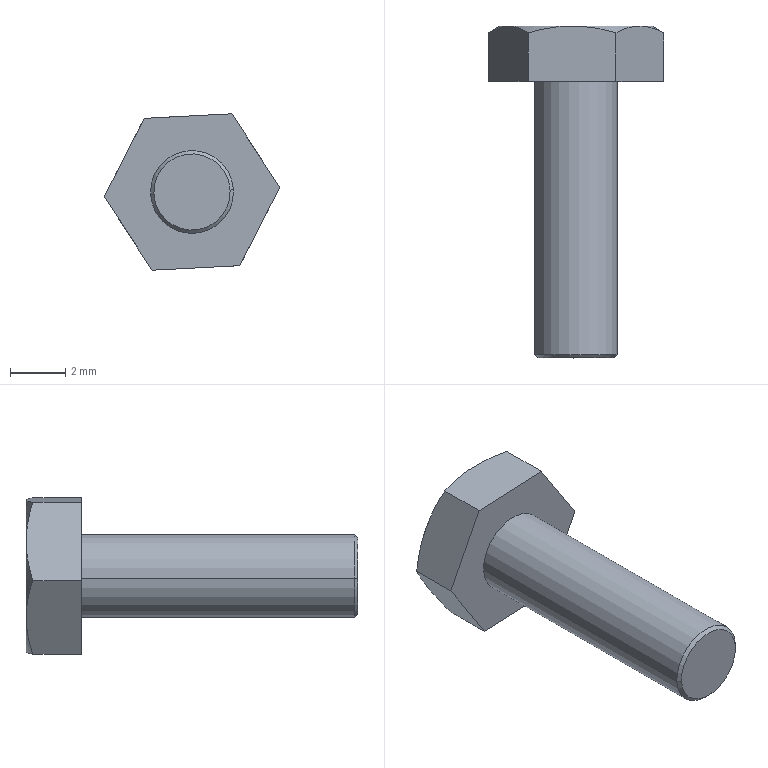Component | SolidWorks | TRCBASHexagonThroughHoleBolt[TRCBAS3-10]-1 | 1 solid | 20 faces | box 6.34 x 12 x 5.66 mm | volume 123 mm3 | cone 9 | plane 9 | cylinder 2 | commonest cylinder face diameters 3 x2
STEP:
#1=COLOUR_RGB('',0.7922,0.8196,0.9333);
#2=FILL_AREA_STYLE_COLOUR('',#1);
#3=FILL_AREA_STYLE('',(#2));
#4=SURFACE_STYLE_FILL_AREA(#3);
#5=SURFACE_SIDE_STYLE('',(#4));
#6=SURFACE_STYLE_USAGE(.BOTH.,#5);
#7=PRESENTATION_STYLE_ASSIGNMENT((#6));
#8=CARTESIAN_POINT('',(2.505,-3.607,-10.617));
#9=VERTEX_POINT('',#8);
#10=CARTESIAN_POINT('',(2.397,-3.607,-10.623));
#11=VERTEX_POINT('',#10);
#12=CARTESIAN_POINT('',(2.451,-3.607,-10.62));
#13=DIRECTION('',(0.,-1.,-0.));
#14=DIRECTION('',(0.9987,0.,0.05162));
#15=AXIS2_PLACEMENT_3D('',#12,#13,#14);
#16=CIRCLE('',#15,0.05433);
#17=EDGE_CURVE('',#9,#11,#16,.T.);
#18=ORIENTED_EDGE('',*,*,#17,.F.);
#19=CARTESIAN_POINT('',(2.51,-3.602,-10.617));
#20=VERTEX_POINT('',#19);
#21=CARTESIAN_POINT('',(2.51,-3.602,-10.617));
#22=DIRECTION('',(0.7062,0.7071,0.0365));
#23=VECTOR('',#22,39.37);
#24=LINE('',#21,#23);
#25=EDGE_CURVE('',#9,#20,#24,.T.);
#26=ORIENTED_EDGE('',*,*,#25,.T.);
#27=CARTESIAN_POINT('',(2.392,-3.602,-10.623));
#28=VERTEX_POINT('',#27);
#29=CARTESIAN_POINT('',(2.451,-3.602,-10.62));
#30=DIRECTION('',(-0.,1.,-0.));
#31=DIRECTION('',(0.9987,0.,0.05162));
#32=AXIS2_PLACEMENT_3D('',#29,#30,#31);
#33=CIRCLE('',#32,0.05906);
#34=EDGE_CURVE('',#28,#20,#33,.T.);
#35=ORIENTED_EDGE('',*,*,#34,.F.);
#36=CARTESIAN_POINT('',(2.392,-3.602,-10.623));
#37=DIRECTION('',(-0.7062,0.7071,-0.0365));
#38=VECTOR('',#37,39.37);
#39=LINE('',#36,#38);
#40=EDGE_CURVE('',#11,#28,#39,.T.);
#41=ORIENTED_EDGE('',*,*,#40,.F.);
#42=EDGE_LOOP('',(#18,#26,#35,#41));
#43=FACE_OUTER_BOUND('',#42,.T.);
#44=CARTESIAN_POINT('',(2.451,-3.602,-10.62));
#45=DIRECTION('',(-0.,1.,-0.));
#46=DIRECTION('',(-0.9987,0.,-0.05162));
#47=AXIS2_PLACEMENT_3D('',#44,#45,#46);
#48=CONICAL_SURFACE('',#47,0.05906,0.7854);
#49=ADVANCED_FACE('',(#43),#48,.T.);
#50=CARTESIAN_POINT('',(2.559,-3.134,-10.614));
#51=VERTEX_POINT('',#50);
#52=CARTESIAN_POINT('',(2.547,-3.134,-10.669));
#53=VERTEX_POINT('',#52);
#54=CARTESIAN_POINT('',(2.451,-3.134,-10.62));
#55=DIRECTION('',(-0.,1.,0.));
#56=DIRECTION('',(-0.9987,0.,-0.05162));
#57=AXIS2_PLACEMENT_3D('',#54,#55,#56);
#58=CIRCLE('',#57,0.1083);
#59=EDGE_CURVE('',#51,#53,#58,.T.);
#60=ORIENTED_EDGE('',*,*,#59,.F.);
#61=CARTESIAN_POINT('',(2.576,-3.144,-10.614));
#62=VERTEX_POINT('',#61);
#63=CARTESIAN_POINT('',(2.559,-3.134,-10.614));
#64=DIRECTION('',(0.8649,-0.5,0.0447));
#65=VECTOR('',#64,39.37);
#66=LINE('',#63,#65);
#67=EDGE_CURVE('',#51,#62,#66,.T.);
#68=ORIENTED_EDGE('',*,*,#67,.T.);
#69=CARTESIAN_POINT('',(2.547,-3.134,-10.669));
#70=CARTESIAN_POINT('',(2.552,-3.134,-10.66));
#71=CARTESIAN_POINT('',(2.557,-3.135,-10.65));
#72=CARTESIAN_POINT('',(2.567,-3.138,-10.632));
#73=CARTESIAN_POINT('',(2.571,-3.141,-10.623));
#74=CARTESIAN_POINT('',(2.576,-3.144,-10.614));
#75=B_SPLINE_CURVE_WITH_KNOTS('',3,(#69,#70,#71,#72,#73,#74),.UNSPECIFIED.,.F.,.F.,(4,2,4),(0.001607,0.002407,0.003207),.UNSPECIFIED.);
#76=EDGE_CURVE('',#53,#62,#75,.T.);
#77=ORIENTED_EDGE('',*,*,#76,.F.);
#78=EDGE_LOOP('',(#60,#68,#77));
#79=FACE_OUTER_BOUND('',#78,.T.);
#80=CARTESIAN_POINT('',(2.451,-3.134,-10.62));
#81=DIRECTION('',(0.,-1.,-0.));
#82=DIRECTION('',(0.9987,0.,0.05162));
#83=AXIS2_PLACEMENT_3D('',#80,#81,#82);
#84=CONICAL_SURFACE('',#83,0.1083,1.047);
#85=ADVANCED_FACE('',(#79),#84,.T.);
#86=ORIENTED_EDGE('',*,*,#34,.T.);
#87=CARTESIAN_POINT('',(2.51,-3.213,-10.617));
#88=VERTEX_POINT('',#87);
#89=CARTESIAN_POINT('',(2.51,-3.134,-10.617));
#90=DIRECTION('',(-0.,1.,0.));
#91=VECTOR('',#90,39.37);
#92=LINE('',#89,#91);
#93=EDGE_CURVE('',#20,#88,#92,.T.);
#94=ORIENTED_EDGE('',*,*,#93,.T.);
#95=CARTESIAN_POINT('',(2.392,-3.213,-10.623));
#96=VERTEX_POINT('',#95);
#97=CARTESIAN_POINT('',(2.451,-3.213,-10.62));
#98=DIRECTION('',(-0.,1.,0.));
#99=DIRECTION('',(-0.9987,0.,-0.05162));
#100=AXIS2_PLACEMENT_3D('',#97,#98,#99);
#101=CIRCLE('',#100,0.05906);
#102=EDGE_CURVE('',#96,#88,#101,.T.);
#103=ORIENTED_EDGE('',*,*,#102,.F.);
#104=CARTESIAN_POINT('',(2.392,-3.134,-10.623));
#105=DIRECTION('',(-0.,1.,0.));
#106=VECTOR('',#105,39.37);
#107=LINE('',#104,#106);
#108=EDGE_CURVE('',#28,#96,#107,.T.);
#109=ORIENTED_EDGE('',*,*,#108,.F.);
#110=EDGE_LOOP('',(#86,#94,#103,#109));
#111=FACE_OUTER_BOUND('',#110,.T.);
#112=CARTESIAN_POINT('',(2.451,-3.134,-10.62));
#113=DIRECTION('',(-0.,1.,0.));
#114=DIRECTION('',(-0.9987,0.,-0.05162));
#115=AXIS2_PLACEMENT_3D('',#112,#113,#114);
#116=CYLINDRICAL_SURFACE('',#115,0.05906);
#117=ADVANCED_FACE('',(#111),#116,.T.);
#118=CARTESIAN_POINT('',(2.576,-3.213,-10.614));
#119=VERTEX_POINT('',#118);
#120=CARTESIAN_POINT('',(2.576,-3.213,-10.614));
#121=DIRECTION('',(-0.,1.,0.));
#122=VECTOR('',#121,39.37);
#123=LINE('',#120,#122);
#124=EDGE_CURVE('',#119,#62,#123,.T.);
#125=ORIENTED_EDGE('',*,*,#124,.T.);
#126=CARTESIAN_POINT('',(2.542,-3.134,-10.561));
#127=VERTEX_POINT('',#126);
#128=CARTESIAN_POINT('',(2.576,-3.144,-10.614));
#129=CARTESIAN_POINT('',(2.565,-3.138,-10.596));
#130=CARTESIAN_POINT('',(2.553,-3.134,-10.579));
#131=CARTESIAN_POINT('',(2.542,-3.134,-10.561));
#132=B_SPLINE_CURVE_WITH_KNOTS('',3,(#128,#129,#130,#131),.UNSPECIFIED.,.F.,.F.,(4,4),(0.00000024,0.001607),.UNSPECIFIED.);
#133=EDGE_CURVE('',#62,#127,#132,.T.);
#134=ORIENTED_EDGE('',*,*,#133,.T.);
#135=CARTESIAN_POINT('',(2.508,-3.144,-10.509));
#136=VERTEX_POINT('',#135);
#137=CARTESIAN_POINT('',(2.542,-3.134,-10.561));
#138=CARTESIAN_POINT('',(2.536,-3.134,-10.552));
#139=CARTESIAN_POINT('',(2.53,-3.135,-10.543));
#140=CARTESIAN_POINT('',(2.519,-3.138,-10.526));
#141=CARTESIAN_POINT('',(2.513,-3.141,-10.517));
#142=CARTESIAN_POINT('',(2.508,-3.144,-10.509));
#143=B_SPLINE_CURVE_WITH_KNOTS('',3,(#137,#138,#139,#140,#141,#142),.UNSPECIFIED.,.F.,.F.,(4,2,4),(0.001607,0.002407,0.003207),.UNSPECIFIED.);
#144=EDGE_CURVE('',#127,#136,#143,.T.);
#145=ORIENTED_EDGE('',*,*,#144,.T.);
#146=CARTESIAN_POINT('',(2.508,-3.213,-10.509));
#147=VERTEX_POINT('',#146);
#148=CARTESIAN_POINT('',(2.508,-3.213,-10.509));
#149=DIRECTION('',(-0.,1.,0.));
#150=VECTOR('',#149,39.37);
#151=LINE('',#148,#150);
#152=EDGE_CURVE('',#147,#136,#151,.T.);
#153=ORIENTED_EDGE('',*,*,#152,.F.);
#154=CARTESIAN_POINT('',(2.508,-3.213,-10.509));
#155=DIRECTION('',(0.544,0.,-0.8391));
#156=VECTOR('',#155,39.37);
#157=LINE('',#154,#156);
#158=EDGE_CURVE('',#147,#119,#157,.T.);
#159=ORIENTED_EDGE('',*,*,#158,.T.);
#160=EDGE_LOOP('',(#125,#134,#145,#153,#159));
#161=FACE_OUTER_BOUND('',#160,.T.);
#162=CARTESIAN_POINT('',(2.508,-3.213,-10.509));
#163=DIRECTION('',(0.8391,0.,0.544));
#164=DIRECTION('',(0.544,0.,-0.8391));
#165=AXIS2_PLACEMENT_3D('',#162,#163,#164);
#166=PLANE('',#165);
#167=ADVANCED_FACE('',(#161),#166,.T.);
#168=ORIENTED_EDGE('',*,*,#152,.T.);
#169=CARTESIAN_POINT('',(2.445,-3.134,-10.512));
#170=VERTEX_POINT('',#169);
#171=CARTESIAN_POINT('',(2.508,-3.144,-10.509));
#172=CARTESIAN_POINT('',(2.498,-3.141,-10.509));
#173=CARTESIAN_POINT('',(2.488,-3.139,-10.51));
#174=CARTESIAN_POINT('',(2.467,-3.135,-10.511));
#175=CARTESIAN_POINT('',(2.456,-3.134,-10.511));
#176=CARTESIAN_POINT('',(2.445,-3.134,-10.512));
#177=B_SPLINE_CURVE_WITH_KNOTS('',3,(#171,#172,#173,#174,#175,#176),.UNSPECIFIED.,.F.,.F.,(4,2,4),(0.008159,0.008963,0.009767),.UNSPECIFIED.);
#178=EDGE_CURVE('',#136,#170,#177,.T.);
#179=ORIENTED_EDGE('',*,*,#178,.T.);
#180=CARTESIAN_POINT('',(2.383,-3.144,-10.515));
#181=VERTEX_POINT('',#180);
#182=CARTESIAN_POINT('',(2.445,-3.134,-10.512));
#183=CARTESIAN_POINT('',(2.435,-3.134,-10.513));
#184=CARTESIAN_POINT('',(2.424,-3.135,-10.513));
#185=CARTESIAN_POINT('',(2.404,-3.138,-10.514));
#186=CARTESIAN_POINT('',(2.393,-3.141,-10.515));
#187=CARTESIAN_POINT('',(2.383,-3.144,-10.515));
#188=B_SPLINE_CURVE_WITH_KNOTS('',3,(#182,#183,#184,#185,#186,#187),.UNSPECIFIED.,.F.,.F.,(4,2,4),(0.009767,0.01057,0.01137),.UNSPECIFIED.);
#189=EDGE_CURVE('',#170,#181,#188,.T.);
#190=ORIENTED_EDGE('',*,*,#189,.T.);
#191=CARTESIAN_POINT('',(2.383,-3.213,-10.515));
#192=VERTEX_POINT('',#191);
#193=CARTESIAN_POINT('',(2.383,-3.213,-10.515));
#194=DIRECTION('',(-0.,1.,0.));
#195=VECTOR('',#194,39.37);
#196=LINE('',#193,#195);
#197=EDGE_CURVE('',#192,#181,#196,.T.);
#198=ORIENTED_EDGE('',*,*,#197,.F.);
#199=CARTESIAN_POINT('',(2.383,-3.213,-10.515));
#200=DIRECTION('',(0.9987,0.,0.05162));
#201=VECTOR('',#200,39.37);
#202=LINE('',#199,#201);
#203=EDGE_CURVE('',#192,#147,#202,.T.);
#204=ORIENTED_EDGE('',*,*,#203,.T.);
#205=EDGE_LOOP('',(#168,#179,#190,#198,#204));
#206=FACE_OUTER_BOUND('',#205,.T.);
#207=CARTESIAN_POINT('',(2.383,-3.213,-10.515));
#208=DIRECTION('',(-0.05162,-0.,0.9987));
#209=DIRECTION('',(0.9987,-0.,0.05162));
#210=AXIS2_PLACEMENT_3D('',#207,#208,#209);
#211=PLANE('',#210);
#212=ADVANCED_FACE('',(#206),#211,.T.);
#213=ORIENTED_EDGE('',*,*,#197,.T.);
#214=CARTESIAN_POINT('',(2.355,-3.134,-10.571));
#215=VERTEX_POINT('',#214);
#216=CARTESIAN_POINT('',(2.383,-3.144,-10.515));
#217=CARTESIAN_POINT('',(2.374,-3.138,-10.533));
#218=CARTESIAN_POINT('',(2.364,-3.134,-10.552));
#219=CARTESIAN_POINT('',(2.355,-3.134,-10.571));
#220=B_SPLINE_CURVE_WITH_KNOTS('',3,(#216,#217,#218,#219),.UNSPECIFIED.,.F.,.F.,(4,4),(0.00000024,0.001607),.UNSPECIFIED.);
#221=EDGE_CURVE('',#181,#215,#220,.T.);
#222=ORIENTED_EDGE('',*,*,#221,.T.);
#223=CARTESIAN_POINT('',(2.326,-3.144,-10.627));
#224=VERTEX_POINT('',#223);
#225=CARTESIAN_POINT('',(2.355,-3.134,-10.571));
#226=CARTESIAN_POINT('',(2.35,-3.134,-10.58));
#227=CARTESIAN_POINT('',(2.345,-3.135,-10.59));
#228=CARTESIAN_POINT('',(2.336,-3.138,-10.608));
#229=CARTESIAN_POINT('',(2.331,-3.141,-10.617));
#230=CARTESIAN_POINT('',(2.326,-3.144,-10.627));
#231=B_SPLINE_CURVE_WITH_KNOTS('',3,(#225,#226,#227,#228,#229,#230),.UNSPECIFIED.,.F.,.F.,(4,2,4),(0.001607,0.002407,0.003207),.UNSPECIFIED.);
#232=EDGE_CURVE('',#215,#224,#231,.T.);
#233=ORIENTED_EDGE('',*,*,#232,.T.);
#234=CARTESIAN_POINT('',(2.326,-3.213,-10.627));
#235=VERTEX_POINT('',#234);
#236=CARTESIAN_POINT('',(2.326,-3.213,-10.627));
#237=DIRECTION('',(-0.,1.,0.));
#238=VECTOR('',#237,39.37);
#239=LINE('',#236,#238);
#240=EDGE_CURVE('',#235,#224,#239,.T.);
#241=ORIENTED_EDGE('',*,*,#240,.F.);
#242=CARTESIAN_POINT('',(2.326,-3.213,-10.627));
#243=DIRECTION('',(0.4546,0.,0.8907));
#244=VECTOR('',#243,39.37);
#245=LINE('',#242,#244);
#246=EDGE_CURVE('',#235,#192,#245,.T.);
#247=ORIENTED_EDGE('',*,*,#246,.T.);
#248=EDGE_LOOP('',(#213,#222,#233,#241,#247));
#249=FACE_OUTER_BOUND('',#248,.T.);
#250=CARTESIAN_POINT('',(2.326,-3.213,-10.627));
#251=DIRECTION('',(-0.8907,-0.,0.4546));
#252=DIRECTION('',(0.4546,-0.,0.8907));
#253=AXIS2_PLACEMENT_3D('',#250,#251,#252);
#254=PLANE('',#253);
#255=ADVANCED_FACE('',(#249),#254,.T.);
#256=ORIENTED_EDGE('',*,*,#240,.T.);
#257=CARTESIAN_POINT('',(2.36,-3.134,-10.679));
#258=VERTEX_POINT('',#257);
#259=CARTESIAN_POINT('',(2.326,-3.144,-10.627));
#260=CARTESIAN_POINT('',(2.337,-3.138,-10.644));
#261=CARTESIAN_POINT('',(2.349,-3.134,-10.661));
#262=CARTESIAN_POINT('',(2.36,-3.134,-10.679));
#263=B_SPLINE_CURVE_WITH_KNOTS('',3,(#259,#260,#261,#262),.UNSPECIFIED.,.F.,.F.,(4,4),(0.00000024,0.001607),.UNSPECIFIED.);
#264=EDGE_CURVE('',#224,#258,#263,.T.);
#265=ORIENTED_EDGE('',*,*,#264,.T.);
#266=CARTESIAN_POINT('',(2.394,-3.144,-10.731));
#267=VERTEX_POINT('',#266);
#268=CARTESIAN_POINT('',(2.36,-3.134,-10.679));
#269=CARTESIAN_POINT('',(2.366,-3.134,-10.688));
#270=CARTESIAN_POINT('',(2.372,-3.135,-10.697));
#271=CARTESIAN_POINT('',(2.383,-3.138,-10.714));
#272=CARTESIAN_POINT('',(2.389,-3.141,-10.723));
#273=CARTESIAN_POINT('',(2.394,-3.144,-10.731));
#274=B_SPLINE_CURVE_WITH_KNOTS('',3,(#268,#269,#270,#271,#272,#273),.UNSPECIFIED.,.F.,.F.,(4,2,4),(0.001607,0.002407,0.003207),.UNSPECIFIED.);
#275=EDGE_CURVE('',#258,#267,#274,.T.);
#276=ORIENTED_EDGE('',*,*,#275,.T.);
#277=CARTESIAN_POINT('',(2.394,-3.213,-10.731));
#278=VERTEX_POINT('',#277);
#279=CARTESIAN_POINT('',(2.394,-3.213,-10.731));
#280=DIRECTION('',(-0.,1.,0.));
#281=VECTOR('',#280,39.37);
#282=LINE('',#279,#281);
#283=EDGE_CURVE('',#278,#267,#282,.T.);
#284=ORIENTED_EDGE('',*,*,#283,.F.);
#285=CARTESIAN_POINT('',(2.394,-3.213,-10.731));
#286=DIRECTION('',(-0.544,-0.,0.8391));
#287=VECTOR('',#286,39.37);
#288=LINE('',#285,#287);
#289=EDGE_CURVE('',#278,#235,#288,.T.);
#290=ORIENTED_EDGE('',*,*,#289,.T.);
#291=EDGE_LOOP('',(#256,#265,#276,#284,#290));
#292=FACE_OUTER_BOUND('',#291,.T.);
#293=CARTESIAN_POINT('',(2.394,-3.213,-10.731));
#294=DIRECTION('',(-0.8391,-0.,-0.544));
#295=DIRECTION('',(-0.544,-0.,0.8391));
#296=AXIS2_PLACEMENT_3D('',#293,#294,#295);
#297=PLANE('',#296);
#298=ADVANCED_FACE('',(#292),#297,.T.);
#299=ORIENTED_EDGE('',*,*,#283,.T.);
#300=CARTESIAN_POINT('',(2.457,-3.134,-10.728));
#301=VERTEX_POINT('',#300);
#302=CARTESIAN_POINT('',(2.394,-3.144,-10.731));
#303=CARTESIAN_POINT('',(2.404,-3.141,-10.731));
#304=CARTESIAN_POINT('',(2.415,-3.138,-10.73));
#305=CARTESIAN_POINT('',(2.436,-3.135,-10.729));
#306=CARTESIAN_POINT('',(2.446,-3.134,-10.729));
#307=CARTESIAN_POINT('',(2.457,-3.134,-10.728));
#308=B_SPLINE_CURVE_WITH_KNOTS('',3,(#302,#303,#304,#305,#306,#307),.UNSPECIFIED.,.F.,.F.,(4,2,4),(0.002918,0.003721,0.004525),.UNSPECIFIED.);
#309=EDGE_CURVE('',#267,#301,#308,.T.);
#310=ORIENTED_EDGE('',*,*,#309,.T.);
#311=CARTESIAN_POINT('',(2.519,-3.144,-10.725));
#312=VERTEX_POINT('',#311);
#313=CARTESIAN_POINT('',(2.457,-3.134,-10.728));
#314=CARTESIAN_POINT('',(2.467,-3.134,-10.728));
#315=CARTESIAN_POINT('',(2.478,-3.135,-10.727));
#316=CARTESIAN_POINT('',(2.499,-3.139,-10.726));
#317=CARTESIAN_POINT('',(2.509,-3.141,-10.725));
#318=CARTESIAN_POINT('',(2.519,-3.144,-10.725));
#319=B_SPLINE_CURVE_WITH_KNOTS('',3,(#313,#314,#315,#316,#317,#318),.UNSPECIFIED.,.F.,.F.,(4,2,4),(0.004525,0.005329,0.006133),.UNSPECIFIED.);
#320=EDGE_CURVE('',#301,#312,#319,.T.);
#321=ORIENTED_EDGE('',*,*,#320,.T.);
#322=CARTESIAN_POINT('',(2.519,-3.213,-10.725));
#323=VERTEX_POINT('',#322);
#324=CARTESIAN_POINT('',(2.519,-3.213,-10.725));
#325=DIRECTION('',(-0.,1.,0.));
#326=VECTOR('',#325,39.37);
#327=LINE('',#324,#326);
#328=EDGE_CURVE('',#323,#312,#327,.T.);
#329=ORIENTED_EDGE('',*,*,#328,.F.);
#330=CARTESIAN_POINT('',(2.519,-3.213,-10.725));
#331=DIRECTION('',(-0.9987,-0.,-0.05162));
#332=VECTOR('',#331,39.37);
#333=LINE('',#330,#332);
#334=EDGE_CURVE('',#323,#278,#333,.T.);
#335=ORIENTED_EDGE('',*,*,#334,.T.);
#336=EDGE_LOOP('',(#299,#310,#321,#329,#335));
#337=FACE_OUTER_BOUND('',#336,.T.);
#338=CARTESIAN_POINT('',(2.519,-3.213,-10.725));
#339=DIRECTION('',(0.05162,0.,-0.9987));
#340=DIRECTION('',(-0.9987,0.,-0.05162));
#341=AXIS2_PLACEMENT_3D('',#338,#339,#340);
#342=PLANE('',#341);
#343=ADVANCED_FACE('',(#337),#342,.T.);
#344=ORIENTED_EDGE('',*,*,#328,.T.);
#345=CARTESIAN_POINT('',(2.519,-3.144,-10.725));
#346=CARTESIAN_POINT('',(2.528,-3.138,-10.707));
#347=CARTESIAN_POINT('',(2.538,-3.134,-10.688));
#348=CARTESIAN_POINT('',(2.547,-3.134,-10.669));
#349=B_SPLINE_CURVE_WITH_KNOTS('',3,(#345,#346,#347,#348),.UNSPECIFIED.,.F.,.F.,(4,4),(0.00000024,0.001607),.UNSPECIFIED.);
#350=EDGE_CURVE('',#312,#53,#349,.T.);
#351=ORIENTED_EDGE('',*,*,#350,.T.);
#352=ORIENTED_EDGE('',*,*,#76,.T.);
#353=ORIENTED_EDGE('',*,*,#124,.F.);
#354=CARTESIAN_POINT('',(2.576,-3.213,-10.614));
#355=DIRECTION('',(-0.4546,-0.,-0.8907));
#356=VECTOR('',#355,39.37);
#357=LINE('',#354,#356);
#358=EDGE_CURVE('',#119,#323,#357,.T.);
#359=ORIENTED_EDGE('',*,*,#358,.T.);
#360=EDGE_LOOP('',(#344,#351,#352,#353,#359));
#361=FACE_OUTER_BOUND('',#360,.T.);
#362=CARTESIAN_POINT('',(2.576,-3.213,-10.614));
#363=DIRECTION('',(0.8907,0.,-0.4546));
#364=DIRECTION('',(-0.4546,0.,-0.8907));
#365=AXIS2_PLACEMENT_3D('',#362,#363,#364);
#366=PLANE('',#365);
#367=ADVANCED_FACE('',(#361),#366,.T.);
#368=ORIENTED_EDGE('',*,*,#102,.T.);
#369=CARTESIAN_POINT('',(2.451,-3.213,-10.62));
#370=DIRECTION('',(-0.,1.,0.));
#371=DIRECTION('',(-0.9987,0.,-0.05162));
#372=AXIS2_PLACEMENT_3D('',#369,#370,#371);
#373=CIRCLE('',#372,0.05906);
#374=EDGE_CURVE('',#88,#96,#373,.T.);
#375=ORIENTED_EDGE('',*,*,#374,.T.);
#376=EDGE_LOOP('',(#368,#375));
#377=FACE_BOUND('',#376,.T.);
#378=ORIENTED_EDGE('',*,*,#246,.F.);
#379=ORIENTED_EDGE('',*,*,#289,.F.);
#380=ORIENTED_EDGE('',*,*,#334,.F.);
#381=ORIENTED_EDGE('',*,*,#358,.F.);
#382=ORIENTED_EDGE('',*,*,#158,.F.);
#383=ORIENTED_EDGE('',*,*,#203,.F.);
#384=EDGE_LOOP('',(#378,#379,#380,#381,#382,#383));
#385=FACE_OUTER_BOUND('',#384,.T.);
#386=CARTESIAN_POINT('',(2.559,-3.213,-10.614));
#387=DIRECTION('',(0.,-1.,-0.));
#388=DIRECTION('',(0.9987,0.,0.05162));
#389=AXIS2_PLACEMENT_3D('',#386,#387,#388);
#390=PLANE('',#389);
#391=ADVANCED_FACE('',(#377,#385),#390,.T.);
#392=ORIENTED_EDGE('',*,*,#93,.F.);
#393=CARTESIAN_POINT('',(2.451,-3.602,-10.62));
#394=DIRECTION('',(-0.,1.,-0.));
#395=DIRECTION('',(0.9987,0.,0.05162));
#396=AXIS2_PLACEMENT_3D('',#393,#394,#395);
#397=CIRCLE('',#396,0.05906);
#398=EDGE_CURVE('',#20,#28,#397,.T.);
#399=ORIENTED_EDGE('',*,*,#398,.T.);
#400=ORIENTED_EDGE('',*,*,#108,.T.);
#401=ORIENTED_EDGE('',*,*,#374,.F.);
#402=EDGE_LOOP('',(#392,#399,#400,#401));
#403=FACE_OUTER_BOUND('',#402,.T.);
#404=CARTESIAN_POINT('',(2.451,-3.134,-10.62));
#405=DIRECTION('',(-0.,1.,0.));
#406=DIRECTION('',(-0.9987,0.,-0.05162));
#407=AXIS2_PLACEMENT_3D('',#404,#405,#406);
#408=CYLINDRICAL_SURFACE('',#407,0.05906);
#409=ADVANCED_FACE('',(#403),#408,.T.);
#410=CARTESIAN_POINT('',(2.451,-3.607,-10.62));
#411=DIRECTION('',(0.,-1.,-0.));
#412=DIRECTION('',(0.9987,0.,0.05162));
#413=AXIS2_PLACEMENT_3D('',#410,#411,#412);
#414=CIRCLE('',#413,0.05433);
#415=EDGE_CURVE('',#11,#9,#414,.T.);
#416=ORIENTED_EDGE('',*,*,#415,.T.);
#417=ORIENTED_EDGE('',*,*,#17,.T.);
#418=EDGE_LOOP('',(#416,#417));
#419=FACE_OUTER_BOUND('',#418,.T.);
#420=CARTESIAN_POINT('',(2.51,-3.607,-10.617));
#421=DIRECTION('',(0.,-1.,-0.));
#422=DIRECTION('',(0.9987,0.,0.05162));
#423=AXIS2_PLACEMENT_3D('',#420,#421,#422);
#424=PLANE('',#423);
#425=ADVANCED_FACE('',(#419),#424,.T.);
#426=CARTESIAN_POINT('',(2.451,-3.134,-10.62));
#427=DIRECTION('',(-0.,1.,0.));
#428=DIRECTION('',(-0.9987,0.,-0.05162));
#429=AXIS2_PLACEMENT_3D('',#426,#427,#428);
#430=CIRCLE('',#429,0.1083);
#431=EDGE_CURVE('',#258,#215,#430,.T.);
#432=ORIENTED_EDGE('',*,*,#431,.F.);
#433=ORIENTED_EDGE('',*,*,#264,.F.);
#434=ORIENTED_EDGE('',*,*,#232,.F.);
#435=EDGE_LOOP('',(#432,#433,#434));
#436=FACE_OUTER_BOUND('',#435,.T.);
#437=CARTESIAN_POINT('',(2.451,-3.134,-10.62));
#438=DIRECTION('',(0.,-1.,-0.));
#439=DIRECTION('',(0.9987,0.,0.05162));
#440=AXIS2_PLACEMENT_3D('',#437,#438,#439);
#441=CONICAL_SURFACE('',#440,0.1083,1.047);
#442=ADVANCED_FACE('',(#436),#441,.T.);
#443=CARTESIAN_POINT('',(2.451,-3.134,-10.62));
#444=DIRECTION('',(-0.,1.,0.));
#445=DIRECTION('',(-0.9987,0.,-0.05162));
#446=AXIS2_PLACEMENT_3D('',#443,#444,#445);
#447=CIRCLE('',#446,0.1083);
#448=EDGE_CURVE('',#301,#258,#447,.T.);
#449=ORIENTED_EDGE('',*,*,#448,.F.);
#450=ORIENTED_EDGE('',*,*,#309,.F.);
#451=ORIENTED_EDGE('',*,*,#275,.F.);
#452=EDGE_LOOP('',(#449,#450,#451));
#453=FACE_OUTER_BOUND('',#452,.T.);
#454=CARTESIAN_POINT('',(2.451,-3.134,-10.62));
#455=DIRECTION('',(0.,-1.,-0.));
#456=DIRECTION('',(0.9987,0.,0.05162));
#457=AXIS2_PLACEMENT_3D('',#454,#455,#456);
#458=CONICAL_SURFACE('',#457,0.1083,1.047);
#459=ADVANCED_FACE('',(#453),#458,.T.);
#460=CARTESIAN_POINT('',(2.451,-3.134,-10.62));
#461=DIRECTION('',(-0.,1.,0.));
#462=DIRECTION('',(-0.9987,0.,-0.05162));
#463=AXIS2_PLACEMENT_3D('',#460,#461,#462);
#464=CIRCLE('',#463,0.1083);
#465=EDGE_CURVE('',#53,#301,#464,.T.);
#466=ORIENTED_EDGE('',*,*,#465,.F.);
#467=ORIENTED_EDGE('',*,*,#350,.F.);
#468=ORIENTED_EDGE('',*,*,#320,.F.);
#469=EDGE_LOOP('',(#466,#467,#468));
#470=FACE_OUTER_BOUND('',#469,.T.);
#471=CARTESIAN_POINT('',(2.451,-3.134,-10.62));
#472=DIRECTION('',(0.,-1.,-0.));
#473=DIRECTION('',(0.9987,0.,0.05162));
#474=AXIS2_PLACEMENT_3D('',#471,#472,#473);
#475=CONICAL_SURFACE('',#474,0.1083,1.047);
#476=ADVANCED_FACE('',(#470),#475,.T.);
#477=ORIENTED_EDGE('',*,*,#67,.F.);
#478=CARTESIAN_POINT('',(2.451,-3.134,-10.62));
#479=DIRECTION('',(-0.,1.,0.));
#480=DIRECTION('',(-0.9987,0.,-0.05162));
#481=AXIS2_PLACEMENT_3D('',#478,#479,#480);
#482=CIRCLE('',#481,0.1083);
#483=EDGE_CURVE('',#127,#51,#482,.T.);
#484=ORIENTED_EDGE('',*,*,#483,.F.);
#485=ORIENTED_EDGE('',*,*,#133,.F.);
#486=EDGE_LOOP('',(#477,#484,#485));
#487=FACE_OUTER_BOUND('',#486,.T.);
#488=CARTESIAN_POINT('',(2.451,-3.134,-10.62));
#489=DIRECTION('',(0.,-1.,-0.));
#490=DIRECTION('',(0.9987,0.,0.05162));
#491=AXIS2_PLACEMENT_3D('',#488,#489,#490);
#492=CONICAL_SURFACE('',#491,0.1083,1.047);
#493=ADVANCED_FACE('',(#487),#492,.T.);
#494=CARTESIAN_POINT('',(2.451,-3.134,-10.62));
#495=DIRECTION('',(-0.,1.,0.));
#496=DIRECTION('',(-0.9987,0.,-0.05162));
#497=AXIS2_PLACEMENT_3D('',#494,#495,#496);
#498=CIRCLE('',#497,0.1083);
#499=EDGE_CURVE('',#170,#127,#498,.T.);
#500=ORIENTED_EDGE('',*,*,#499,.F.);
#501=ORIENTED_EDGE('',*,*,#178,.F.);
#502=ORIENTED_EDGE('',*,*,#144,.F.);
#503=EDGE_LOOP('',(#500,#501,#502));
#504=FACE_OUTER_BOUND('',#503,.T.);
#505=CARTESIAN_POINT('',(2.451,-3.134,-10.62));
#506=DIRECTION('',(0.,-1.,-0.));
#507=DIRECTION('',(0.9987,0.,0.05162));
#508=AXIS2_PLACEMENT_3D('',#505,#506,#507);
#509=CONICAL_SURFACE('',#508,0.1083,1.047);
#510=ADVANCED_FACE('',(#504),#509,.T.);
#511=CARTESIAN_POINT('',(2.451,-3.134,-10.62));
#512=DIRECTION('',(-0.,1.,0.));
#513=DIRECTION('',(-0.9987,0.,-0.05162));
#514=AXIS2_PLACEMENT_3D('',#511,#512,#513);
#515=CIRCLE('',#514,0.1083);
#516=EDGE_CURVE('',#215,#170,#515,.T.);
#517=ORIENTED_EDGE('',*,*,#516,.F.);
#518=ORIENTED_EDGE('',*,*,#221,.F.);
#519=ORIENTED_EDGE('',*,*,#189,.F.);
#520=EDGE_LOOP('',(#517,#518,#519));
#521=FACE_OUTER_BOUND('',#520,.T.);
#522=CARTESIAN_POINT('',(2.451,-3.134,-10.62));
#523=DIRECTION('',(0.,-1.,-0.));
#524=DIRECTION('',(0.9987,0.,0.05162));
#525=AXIS2_PLACEMENT_3D('',#522,#523,#524);
#526=CONICAL_SURFACE('',#525,0.1083,1.047);
#527=ADVANCED_FACE('',(#521),#526,.T.);
#528=ORIENTED_EDGE('',*,*,#431,.T.);
#529=ORIENTED_EDGE('',*,*,#516,.T.);
#530=ORIENTED_EDGE('',*,*,#499,.T.);
#531=ORIENTED_EDGE('',*,*,#483,.T.);
#532=ORIENTED_EDGE('',*,*,#59,.T.);
#533=ORIENTED_EDGE('',*,*,#465,.T.);
#534=ORIENTED_EDGE('',*,*,#448,.T.);
#535=EDGE_LOOP('',(#528,#529,#530,#531,#532,#533,#534));
#536=FACE_OUTER_BOUND('',#535,.T.);
#537=CARTESIAN_POINT('',(2.559,-3.134,-10.614));
#538=DIRECTION('',(-0.,1.,0.));
#539=DIRECTION('',(-0.9987,-0.,-0.05162));
#540=AXIS2_PLACEMENT_3D('',#537,#538,#539);
#541=PLANE('',#540);
#542=ADVANCED_FACE('',(#536),#541,.T.);
#543=ORIENTED_EDGE('',*,*,#25,.F.);
#544=ORIENTED_EDGE('',*,*,#415,.F.);
#545=ORIENTED_EDGE('',*,*,#40,.T.);
#546=ORIENTED_EDGE('',*,*,#398,.F.);
#547=EDGE_LOOP('',(#543,#544,#545,#546));
#548=FACE_OUTER_BOUND('',#547,.T.);
#549=CARTESIAN_POINT('',(2.451,-3.602,-10.62));
#550=DIRECTION('',(-0.,1.,-0.));
#551=DIRECTION('',(-0.9987,0.,-0.05162));
#552=AXIS2_PLACEMENT_3D('',#549,#550,#551);
#553=CONICAL_SURFACE('',#552,0.05906,0.7854);
#554=ADVANCED_FACE('',(#548),#553,.T.);
#555=CLOSED_SHELL('',(#49,#85,#117,#167,#212,#255,#298,#343,#367,#391,#409,#425,#442,#459,#476,#493,#510,#527,#542,#554));
#556=MANIFOLD_SOLID_BREP('',#555);
#557=STYLED_ITEM('',(#7),#556);
#558=(LENGTH_UNIT()NAMED_UNIT(*)SI_UNIT($,.METRE.));
#559=LENGTH_MEASURE_WITH_UNIT(LENGTH_MEASURE(0.0254),#558);
#560=DIMENSIONAL_EXPONENTS(1.,0.,0.,0.,0.,0.,0.);
#561=(CONVERSION_BASED_UNIT('',#559)LENGTH_UNIT()NAMED_UNIT(#560));
#562=UNCERTAINTY_MEASURE_WITH_UNIT(LENGTH_MEASURE(0.00001),#561,'','');
#563=(NAMED_UNIT(*)PLANE_ANGLE_UNIT()SI_UNIT($,.RADIAN.));
#564=(NAMED_UNIT(*)SI_UNIT($,.STERADIAN.)SOLID_ANGLE_UNIT());
#565=(GEOMETRIC_REPRESENTATION_CONTEXT(3)GLOBAL_UNCERTAINTY_ASSIGNED_CONTEXT((#562))GLOBAL_UNIT_ASSIGNED_CONTEXT((#561,#563,#564))REPRESENTATION_CONTEXT('',''));
#566=MECHANICAL_DESIGN_GEOMETRIC_PRESENTATION_REPRESENTATION('',(#557),#565);
#567=CARTESIAN_POINT('',(0.,0.,0.));
#568=DIRECTION('',(0.,0.,1.));
#569=DIRECTION('',(1.,0.,0.));
#570=AXIS2_PLACEMENT_3D('',#567,#568,#569);
#571=(LENGTH_UNIT()NAMED_UNIT(*)SI_UNIT($,.METRE.));
#572=LENGTH_MEASURE_WITH_UNIT(LENGTH_MEASURE(0.0254),#571);
#573=DIMENSIONAL_EXPONENTS(1.,0.,0.,0.,0.,0.,0.);
#574=(CONVERSION_BASED_UNIT('',#572)LENGTH_UNIT()NAMED_UNIT(#573));
#575=UNCERTAINTY_MEASURE_WITH_UNIT(LENGTH_MEASURE(0.00001),#574,'','');
#576=(NAMED_UNIT(*)PLANE_ANGLE_UNIT()SI_UNIT($,.RADIAN.));
#577=(NAMED_UNIT(*)SI_UNIT($,.STERADIAN.)SOLID_ANGLE_UNIT());
#578=(GEOMETRIC_REPRESENTATION_CONTEXT(3)GLOBAL_UNCERTAINTY_ASSIGNED_CONTEXT((#575))GLOBAL_UNIT_ASSIGNED_CONTEXT((#574,#576,#577))REPRESENTATION_CONTEXT('',''));
#579=ADVANCED_BREP_SHAPE_REPRESENTATION('',(#556,#570),#578);
#580=PRESENTATION_LAYER_ASSIGNMENT('','',(#557));